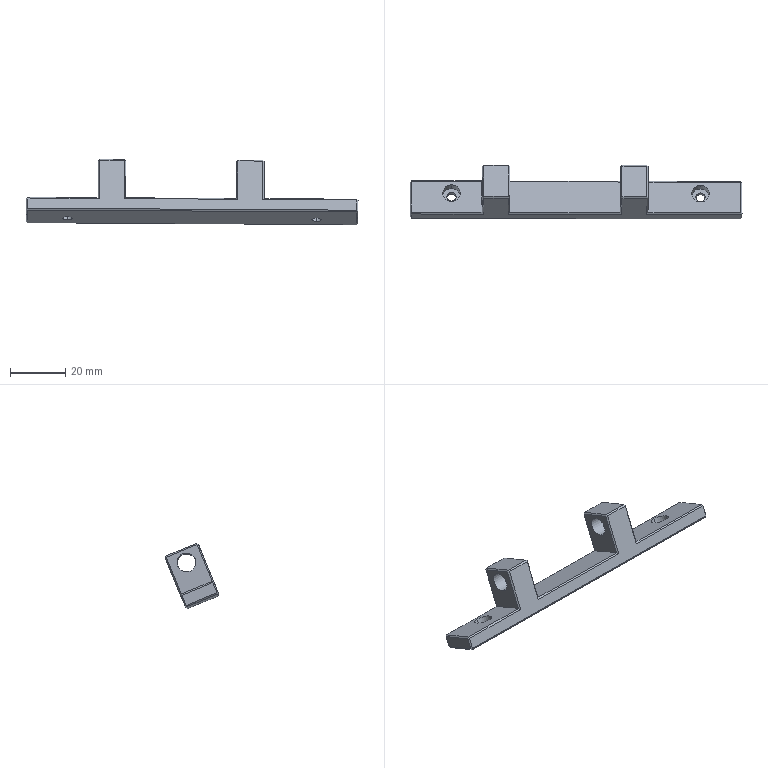Component | SolidWorks | 14-1 | 1 solid | 76 faces | box 120.02 x 19.49 x 23.62 mm | volume 10629 mm3 | plane 64 | cylinder 12 | commonest cylinder face diameters 6.5 x4 3.4 x4 6.8 x4
build123d program:
from build123d import *

# Parameters (mm, degrees)
SKETCH1_W                                       = 13
SKETCH1_H                                       = 120
BOSS_EXTRUDE1_DEPTH                             = 5
SKETCH2_W                                       = 13
SKETCH2_H                                       = 10
BOSS_EXTRUDE2_DEPTH                             = 15
LPATTERN1_COUNT                                 = 2
LPATTERN1_PITCH                                 = 50
M3_HEX_SOCKET_HEAD_CAP_SCREW_CBORE1_D           = 3.4
M3_HEX_SOCKET_HEAD_CAP_SCREW_CBORE1_CBORE_D     = 6.5
M3_HEX_SOCKET_HEAD_CAP_SCREW_CBORE1_CBORE_DEPTH = 3.4
CHAMFER1_SIZE                                   = 0.5


with BuildPart() as part:
    # Sketch1 → Boss-Extrude1 (new body)
    with BuildSketch(Plane.XY):
        Rectangle(SKETCH1_W, SKETCH1_H)
    extrude(amount=BOSS_EXTRUDE1_DEPTH)

    # Sketch2 → Boss-Extrude2 (add)
    with BuildSketch(Plane(origin=(0, 0, 0), x_dir=(-1, 0, 0), z_dir=(0, 0, -1))):
        with Locations((0, 29)):
            Rectangle(SKETCH2_W, SKETCH2_H)
    boss_extrude2 = extrude(amount=BOSS_EXTRUDE2_DEPTH)

    # Sketch3 → M8 Tapped Hole1 (revolve, cut)
    with BuildSketch(Plane(origin=(0, 34, -10), x_dir=(0, 0, 1), z_dir=(1, 0, 0))):
        Polygon((0, 0), (0, 21.793), (3.4, 19.75), (3.4, 0), align=None)
    m8_tapped_hole1 = revolve(axis=Axis((0, 40.35, -10), (0, -1, 0)), mode=Mode.SUBTRACT)

    # LPattern1: Boss-Extrude2, M8 Tapped Hole1 ×2
    with Locations(*[(0, -i * LPATTERN1_PITCH, 0) for i in range(1, LPATTERN1_COUNT)]):
        add(boss_extrude2)
        add(m8_tapped_hole1, mode=Mode.SUBTRACT)

    # M3 Hex Socket Head Cap Screw CBORE1 (through all)
    with Locations(Plane(origin=(0, 0, 0), x_dir=(-1, 0, 0), z_dir=(0, 0, -1))):
        with Locations((1.5, 45), (1.5, -45)):
            CounterBoreHole(M3_HEX_SOCKET_HEAD_CAP_SCREW_CBORE1_D / 2, M3_HEX_SOCKET_HEAD_CAP_SCREW_CBORE1_CBORE_D / 2, M3_HEX_SOCKET_HEAD_CAP_SCREW_CBORE1_CBORE_DEPTH)

    # Chamfer1
    chamfer1_edges = [part.edges().sort_by_distance(p)[0] for p in [
        (-6.5, 60, 2.5),
        (-6.5, 0, 5),
        (-6.5, -60, 2.5),
        (-6.5, -43, 0),
        (-6.5, -26, -7.5),
        (6.5, -26, -7.5),
        (6.5, -21, -15),
        (-6.5, -21, -15),
        (6.5, -16, -7.5),
        (-6.5, -16, -7.5),
        (-6.5, 4, 0),
        (-6.5, 24, -7.5),
        (-6.5, 29, -15),
        (-6.5, 34, -7.5),
        (-6.5, 47, 0),
        (6.5, -60, 2.5),
        (0, -60, 5),
        (6.5, 0, 5),
        (0, 60, 5),
        (6.5, 60, 2.5),
        (0, -60, 0),
        (6.5, -43, 0),
        (0, -26, -15),
        (0, -16, -15),
        (6.5, 4, 0),
        (6.5, 24, -7.5),
        (0, 24, -15),
        (6.5, 29, -15),
        (0, 34, -15),
        (6.5, 34, -7.5),
        (6.5, 47, 0),
        (0, 60, 0),
    ]]
    chamfer(chamfer1_edges, length=CHAMFER1_SIZE)


solid = part.part

# Placed as in the assembly
solid = solid.moved(Location((113.912, -45.575, 442.739), (157.516, -0.3658, 89.992)))